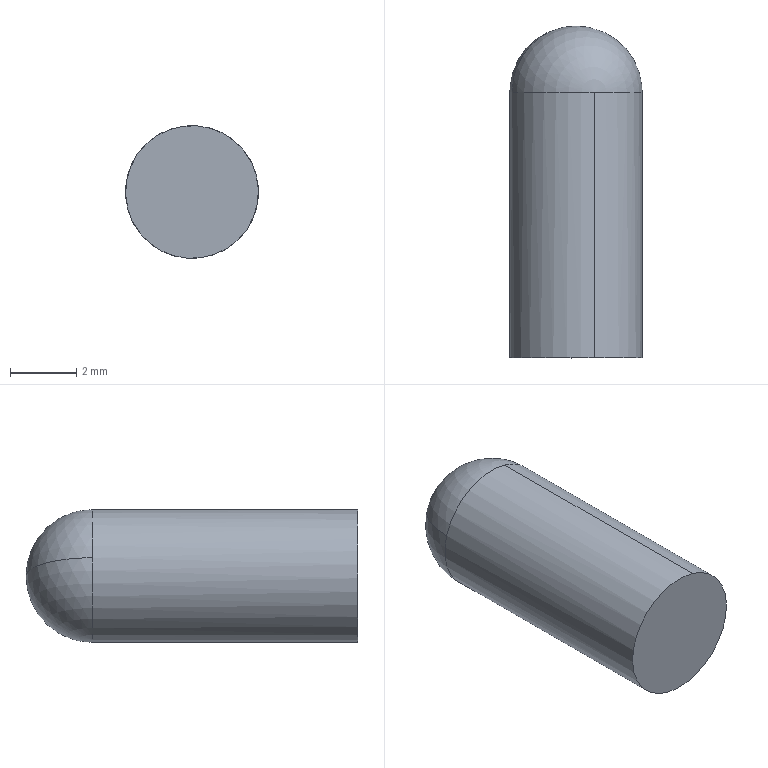Component | SolidWorks | KFQAPP4-P4.00-L4-B4.0-2 | 1 solid | 5 faces | box 4 x 10 x 4 mm | volume 117 mm3 | cylinder 2 | sphere 2 | plane 1 | commonest cylinder face diameters 4 x2
build123d program:
from build123d import *


with BuildPart() as part:
    # Sketch2 → Rotate1 (revolve)
    with BuildSketch(Plane.XY):
        with BuildLine():
            Line((0, 5), (0, -5))
            Line((0, -5), (2, -5))
            Line((2, -5), (2, 3))
            ThreePointArc((2, 3), (1.414, 4.414), (0, 5))
        make_face()
    revolve(axis=Axis((0, 38.331, 0), (0, -1, 0)))


solid = part.part

# Placed as in the assembly
solid = solid.moved(Location((-666.208, -1.092, 131.188), (0, 0, 0)))
STEP:
#1=CARTESIAN_POINT('',(-26.207,-0.2398,5.241));
#2=VERTEX_POINT('',#1);
#3=CARTESIAN_POINT('',(-26.25,-0.2398,5.089));
#4=VERTEX_POINT('',#3);
#5=CARTESIAN_POINT('',(-26.229,-0.2398,5.165));
#6=DIRECTION('',(-0.,1.,-0.));
#7=DIRECTION('',(0.2756,0.,0.9613));
#8=AXIS2_PLACEMENT_3D('',#5,#6,#7);
#9=CIRCLE('',#8,0.07874);
#10=EDGE_CURVE('',#2,#4,#9,.T.);
#11=ORIENTED_EDGE('',*,*,#10,.T.);
#12=CARTESIAN_POINT('',(-26.25,0.07513,5.089));
#13=VERTEX_POINT('',#12);
#14=CARTESIAN_POINT('',(-26.25,1.466,5.089));
#15=DIRECTION('',(-0.,1.,-0.));
#16=VECTOR('',#15,39.37);
#17=LINE('',#14,#16);
#18=EDGE_CURVE('',#4,#13,#17,.T.);
#19=ORIENTED_EDGE('',*,*,#18,.T.);
#20=CARTESIAN_POINT('',(-26.153,0.07513,5.143));
#21=VERTEX_POINT('',#20);
#22=CARTESIAN_POINT('',(-26.229,0.07513,5.165));
#23=DIRECTION('',(-0.,1.,-0.));
#24=DIRECTION('',(0.2756,0.,0.9613));
#25=AXIS2_PLACEMENT_3D('',#22,#23,#24);
#26=CIRCLE('',#25,0.07874);
#27=EDGE_CURVE('',#21,#13,#26,.T.);
#28=ORIENTED_EDGE('',*,*,#27,.F.);
#29=CARTESIAN_POINT('',(-26.207,0.07513,5.241));
#30=VERTEX_POINT('',#29);
#31=CARTESIAN_POINT('',(-26.229,0.07513,5.165));
#32=DIRECTION('',(-0.,1.,-0.));
#33=DIRECTION('',(0.2756,0.,0.9613));
#34=AXIS2_PLACEMENT_3D('',#31,#32,#33);
#35=CIRCLE('',#34,0.07874);
#36=EDGE_CURVE('',#30,#21,#35,.T.);
#37=ORIENTED_EDGE('',*,*,#36,.F.);
#38=CARTESIAN_POINT('',(-26.207,1.466,5.241));
#39=DIRECTION('',(-0.,1.,-0.));
#40=VECTOR('',#39,39.37);
#41=LINE('',#38,#40);
#42=EDGE_CURVE('',#2,#30,#41,.T.);
#43=ORIENTED_EDGE('',*,*,#42,.F.);
#44=EDGE_LOOP('',(#11,#19,#28,#37,#43));
#45=FACE_OUTER_BOUND('',#44,.T.);
#46=CARTESIAN_POINT('',(-26.229,1.466,5.165));
#47=DIRECTION('',(-0.,1.,-0.));
#48=DIRECTION('',(0.2756,0.,0.9613));
#49=AXIS2_PLACEMENT_3D('',#46,#47,#48);
#50=CYLINDRICAL_SURFACE('',#49,0.07874);
#51=ADVANCED_FACE('',(#45),#50,.T.);
#52=ORIENTED_EDGE('',*,*,#27,.T.);
#53=CARTESIAN_POINT('',(-26.304,0.07513,5.187));
#54=VERTEX_POINT('',#53);
#55=CARTESIAN_POINT('',(-26.229,0.07513,5.165));
#56=DIRECTION('',(-0.,1.,-0.));
#57=DIRECTION('',(0.2756,0.,0.9613));
#58=AXIS2_PLACEMENT_3D('',#55,#56,#57);
#59=CIRCLE('',#58,0.07874);
#60=EDGE_CURVE('',#13,#54,#59,.T.);
#61=ORIENTED_EDGE('',*,*,#60,.T.);
#62=CARTESIAN_POINT('',(-26.229,0.1539,5.165));
#63=VERTEX_POINT('',#62);
#64=CARTESIAN_POINT('',(-26.229,0.07513,5.165));
#65=DIRECTION('',(-0.2756,-0.,-0.9613));
#66=DIRECTION('',(-0.9613,0.,0.2756));
#67=AXIS2_PLACEMENT_3D('',#64,#65,#66);
#68=CIRCLE('',#67,0.07874);
#69=EDGE_CURVE('',#54,#63,#68,.T.);
#70=ORIENTED_EDGE('',*,*,#69,.T.);
#71=CARTESIAN_POINT('',(-26.229,0.07513,5.165));
#72=DIRECTION('',(0.2756,0.,0.9613));
#73=DIRECTION('',(0.9613,0.,-0.2756));
#74=AXIS2_PLACEMENT_3D('',#71,#72,#73);
#75=CIRCLE('',#74,0.07874);
#76=EDGE_CURVE('',#21,#63,#75,.T.);
#77=ORIENTED_EDGE('',*,*,#76,.F.);
#78=EDGE_LOOP('',(#52,#61,#70,#77));
#79=FACE_OUTER_BOUND('',#78,.T.);
#80=CARTESIAN_POINT('',(-26.229,0.07513,5.165));
#81=DIRECTION('',(-0.2756,-0.,-0.9613));
#82=DIRECTION('',(0.9613,0.,-0.2756));
#83=AXIS2_PLACEMENT_3D('',#80,#81,#82);
#84=SPHERICAL_SURFACE('',#83,0.07874);
#85=ADVANCED_FACE('',(#79),#84,.T.);
#86=ORIENTED_EDGE('',*,*,#69,.F.);
#87=CARTESIAN_POINT('',(-26.229,0.07513,5.165));
#88=DIRECTION('',(-0.,1.,-0.));
#89=DIRECTION('',(0.2756,0.,0.9613));
#90=AXIS2_PLACEMENT_3D('',#87,#88,#89);
#91=CIRCLE('',#90,0.07874);
#92=EDGE_CURVE('',#54,#30,#91,.T.);
#93=ORIENTED_EDGE('',*,*,#92,.T.);
#94=ORIENTED_EDGE('',*,*,#36,.T.);
#95=ORIENTED_EDGE('',*,*,#76,.T.);
#96=EDGE_LOOP('',(#86,#93,#94,#95));
#97=FACE_OUTER_BOUND('',#96,.T.);
#98=CARTESIAN_POINT('',(-26.229,0.07513,5.165));
#99=DIRECTION('',(-0.2756,-0.,-0.9613));
#100=DIRECTION('',(0.9613,0.,-0.2756));
#101=AXIS2_PLACEMENT_3D('',#98,#99,#100);
#102=SPHERICAL_SURFACE('',#101,0.07874);
#103=ADVANCED_FACE('',(#97),#102,.T.);
#104=ORIENTED_EDGE('',*,*,#10,.F.);
#105=CARTESIAN_POINT('',(-26.229,-0.2398,5.165));
#106=DIRECTION('',(-0.,1.,-0.));
#107=DIRECTION('',(0.2756,0.,0.9613));
#108=AXIS2_PLACEMENT_3D('',#105,#106,#107);
#109=CIRCLE('',#108,0.07874);
#110=EDGE_CURVE('',#4,#2,#109,.T.);
#111=ORIENTED_EDGE('',*,*,#110,.F.);
#112=EDGE_LOOP('',(#104,#111));
#113=FACE_OUTER_BOUND('',#112,.T.);
#114=CARTESIAN_POINT('',(-26.153,-0.2398,5.143));
#115=DIRECTION('',(-0.,1.,-0.));
#116=DIRECTION('',(0.2756,0.,0.9613));
#117=AXIS2_PLACEMENT_3D('',#114,#115,#116);
#118=PLANE('',#117);
#119=ADVANCED_FACE('',(#113),#118,.F.);
#120=ORIENTED_EDGE('',*,*,#18,.F.);
#121=ORIENTED_EDGE('',*,*,#110,.T.);
#122=ORIENTED_EDGE('',*,*,#42,.T.);
#123=ORIENTED_EDGE('',*,*,#92,.F.);
#124=ORIENTED_EDGE('',*,*,#60,.F.);
#125=EDGE_LOOP('',(#120,#121,#122,#123,#124));
#126=FACE_OUTER_BOUND('',#125,.T.);
#127=CARTESIAN_POINT('',(-26.229,1.466,5.165));
#128=DIRECTION('',(-0.,1.,-0.));
#129=DIRECTION('',(0.2756,0.,0.9613));
#130=AXIS2_PLACEMENT_3D('',#127,#128,#129);
#131=CYLINDRICAL_SURFACE('',#130,0.07874);
#132=ADVANCED_FACE('',(#126),#131,.T.);
#133=CLOSED_SHELL('',(#51,#85,#103,#119,#132));
#134=MANIFOLD_SOLID_BREP('',#133);
#135=CARTESIAN_POINT('',(0.,0.,0.));
#136=DIRECTION('',(0.,0.,1.));
#137=DIRECTION('',(1.,0.,0.));
#138=AXIS2_PLACEMENT_3D('',#135,#136,#137);
#139=(LENGTH_UNIT()NAMED_UNIT(*)SI_UNIT($,.METRE.));
#140=LENGTH_MEASURE_WITH_UNIT(LENGTH_MEASURE(0.0254),#139);
#141=DIMENSIONAL_EXPONENTS(1.,0.,0.,0.,0.,0.,0.);
#142=(CONVERSION_BASED_UNIT('',#140)LENGTH_UNIT()NAMED_UNIT(#141));
#143=UNCERTAINTY_MEASURE_WITH_UNIT(LENGTH_MEASURE(0.00001),#142,'','');
#144=(NAMED_UNIT(*)PLANE_ANGLE_UNIT()SI_UNIT($,.RADIAN.));
#145=(NAMED_UNIT(*)SI_UNIT($,.STERADIAN.)SOLID_ANGLE_UNIT());
#146=(GEOMETRIC_REPRESENTATION_CONTEXT(3)GLOBAL_UNCERTAINTY_ASSIGNED_CONTEXT((#143))GLOBAL_UNIT_ASSIGNED_CONTEXT((#142,#144,#145))REPRESENTATION_CONTEXT('',''));
#147=ADVANCED_BREP_SHAPE_REPRESENTATION('',(#134,#138),#146);
#148=COLOUR_RGB('',0.7922,0.8196,0.9333);
#149=FILL_AREA_STYLE_COLOUR('',#148);
#150=FILL_AREA_STYLE('',(#149));
#151=SURFACE_STYLE_FILL_AREA(#150);
#152=SURFACE_SIDE_STYLE('',(#151));
#153=SURFACE_STYLE_USAGE(.BOTH.,#152);
#154=PRESENTATION_STYLE_ASSIGNMENT((#153));
#155=STYLED_ITEM('',(#154),#134);
#156=(LENGTH_UNIT()NAMED_UNIT(*)SI_UNIT($,.METRE.));
#157=LENGTH_MEASURE_WITH_UNIT(LENGTH_MEASURE(0.0254),#156);
#158=DIMENSIONAL_EXPONENTS(1.,0.,0.,0.,0.,0.,0.);
#159=(CONVERSION_BASED_UNIT('',#157)LENGTH_UNIT()NAMED_UNIT(#158));
#160=UNCERTAINTY_MEASURE_WITH_UNIT(LENGTH_MEASURE(0.00001),#159,'','');
#161=(NAMED_UNIT(*)PLANE_ANGLE_UNIT()SI_UNIT($,.RADIAN.));
#162=(NAMED_UNIT(*)SI_UNIT($,.STERADIAN.)SOLID_ANGLE_UNIT());
#163=(GEOMETRIC_REPRESENTATION_CONTEXT(3)GLOBAL_UNCERTAINTY_ASSIGNED_CONTEXT((#160))GLOBAL_UNIT_ASSIGNED_CONTEXT((#159,#161,#162))REPRESENTATION_CONTEXT('',''));
#164=MECHANICAL_DESIGN_GEOMETRIC_PRESENTATION_REPRESENTATION('',(#155),#163);
#165=PRESENTATION_LAYER_ASSIGNMENT('','',(#155));